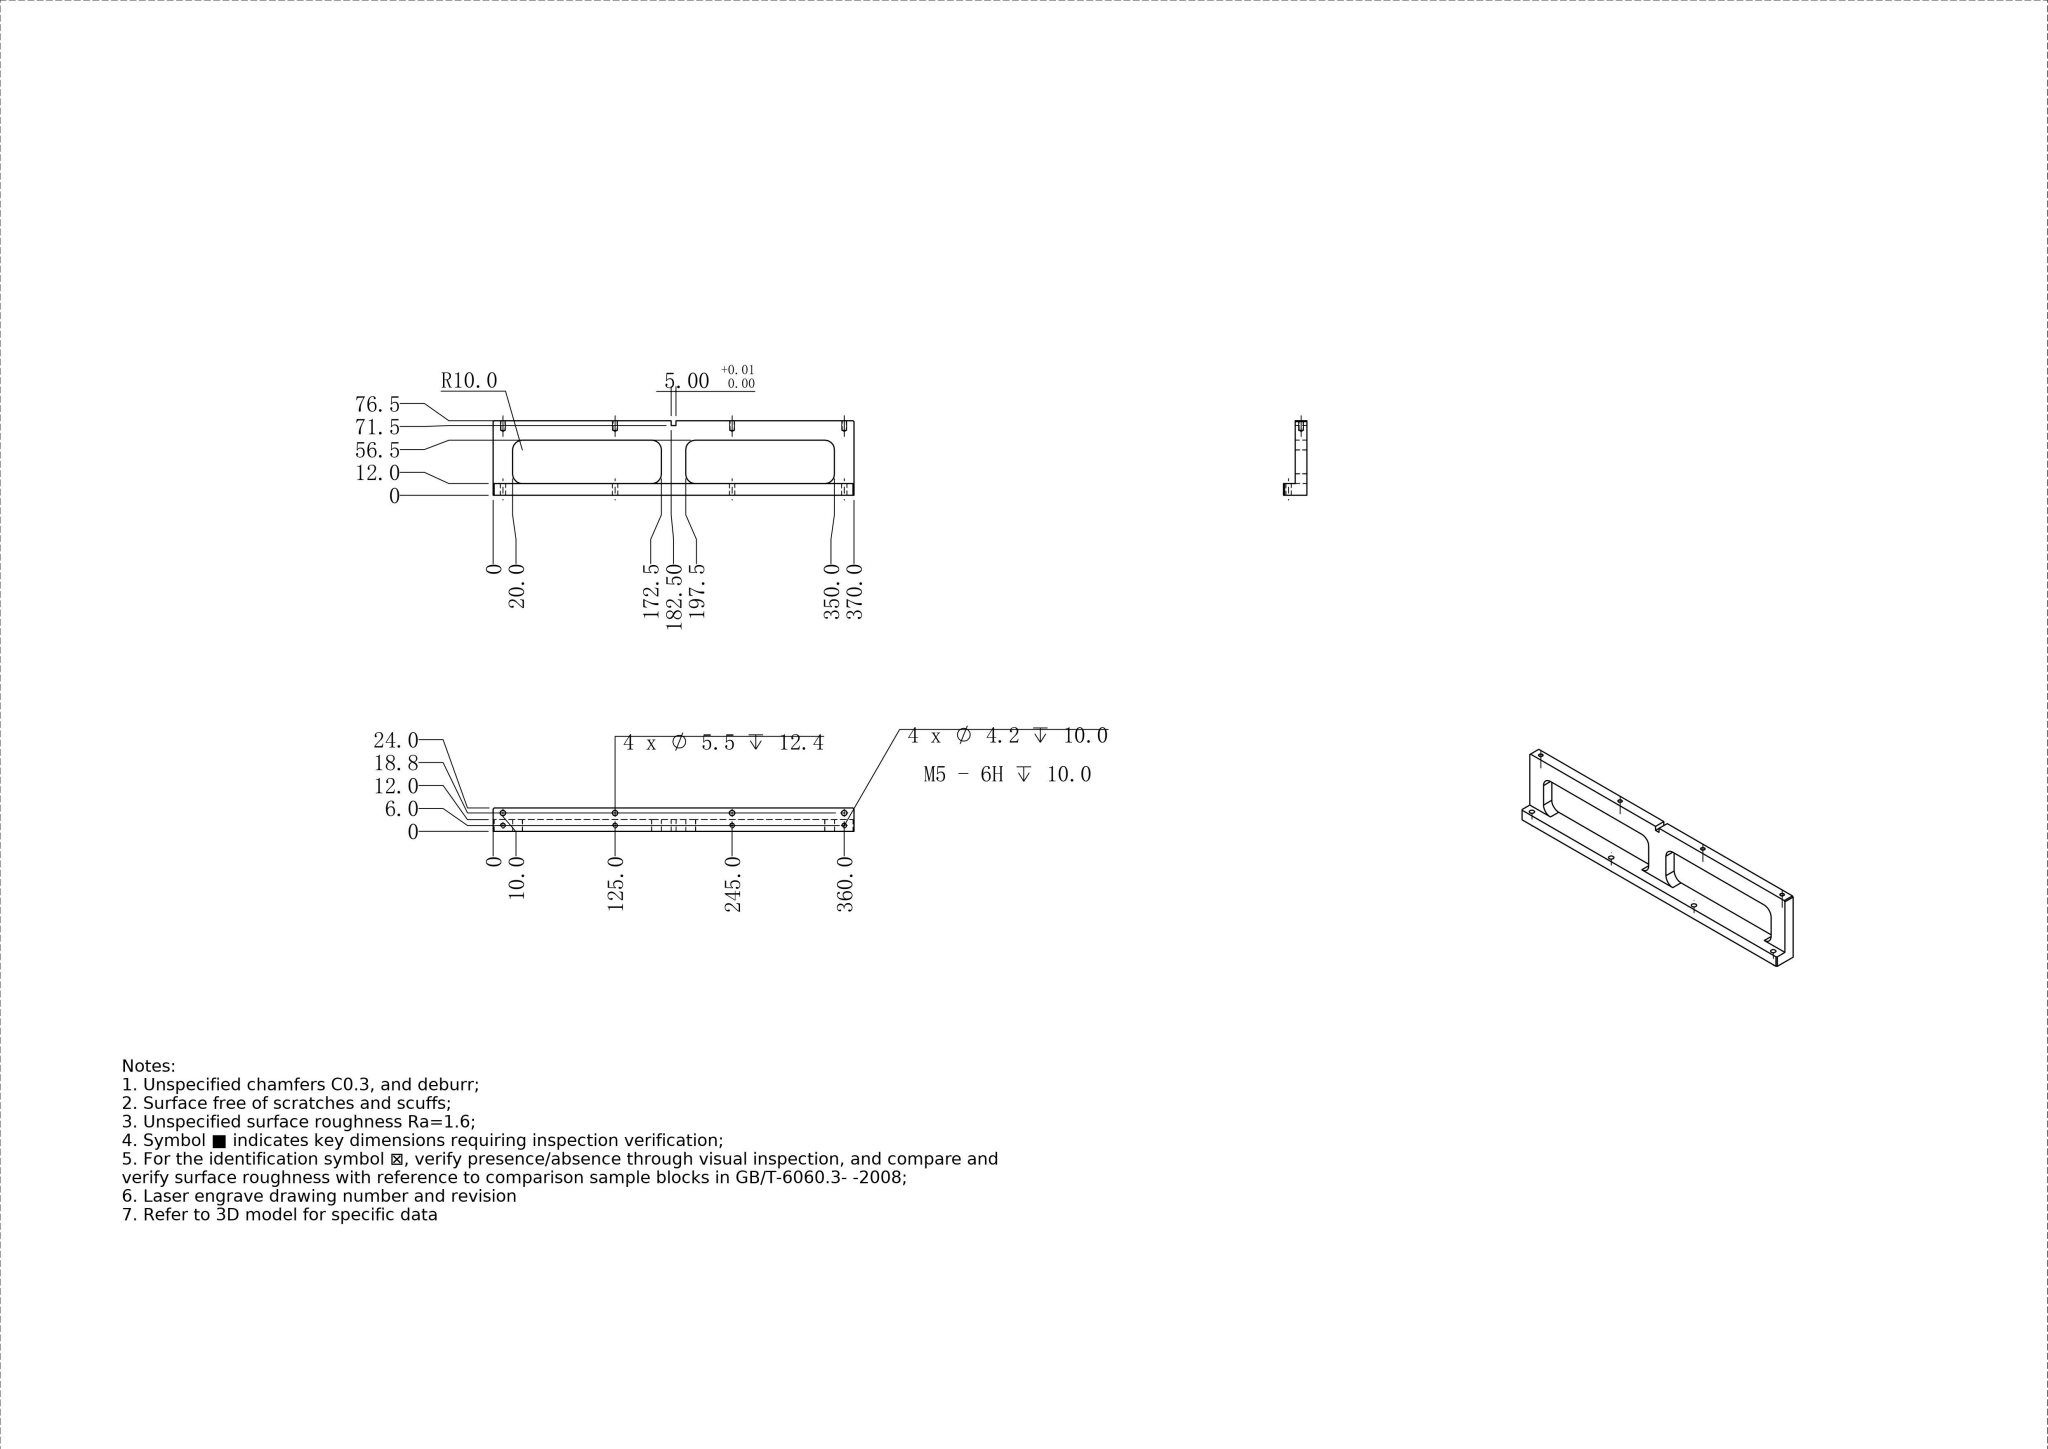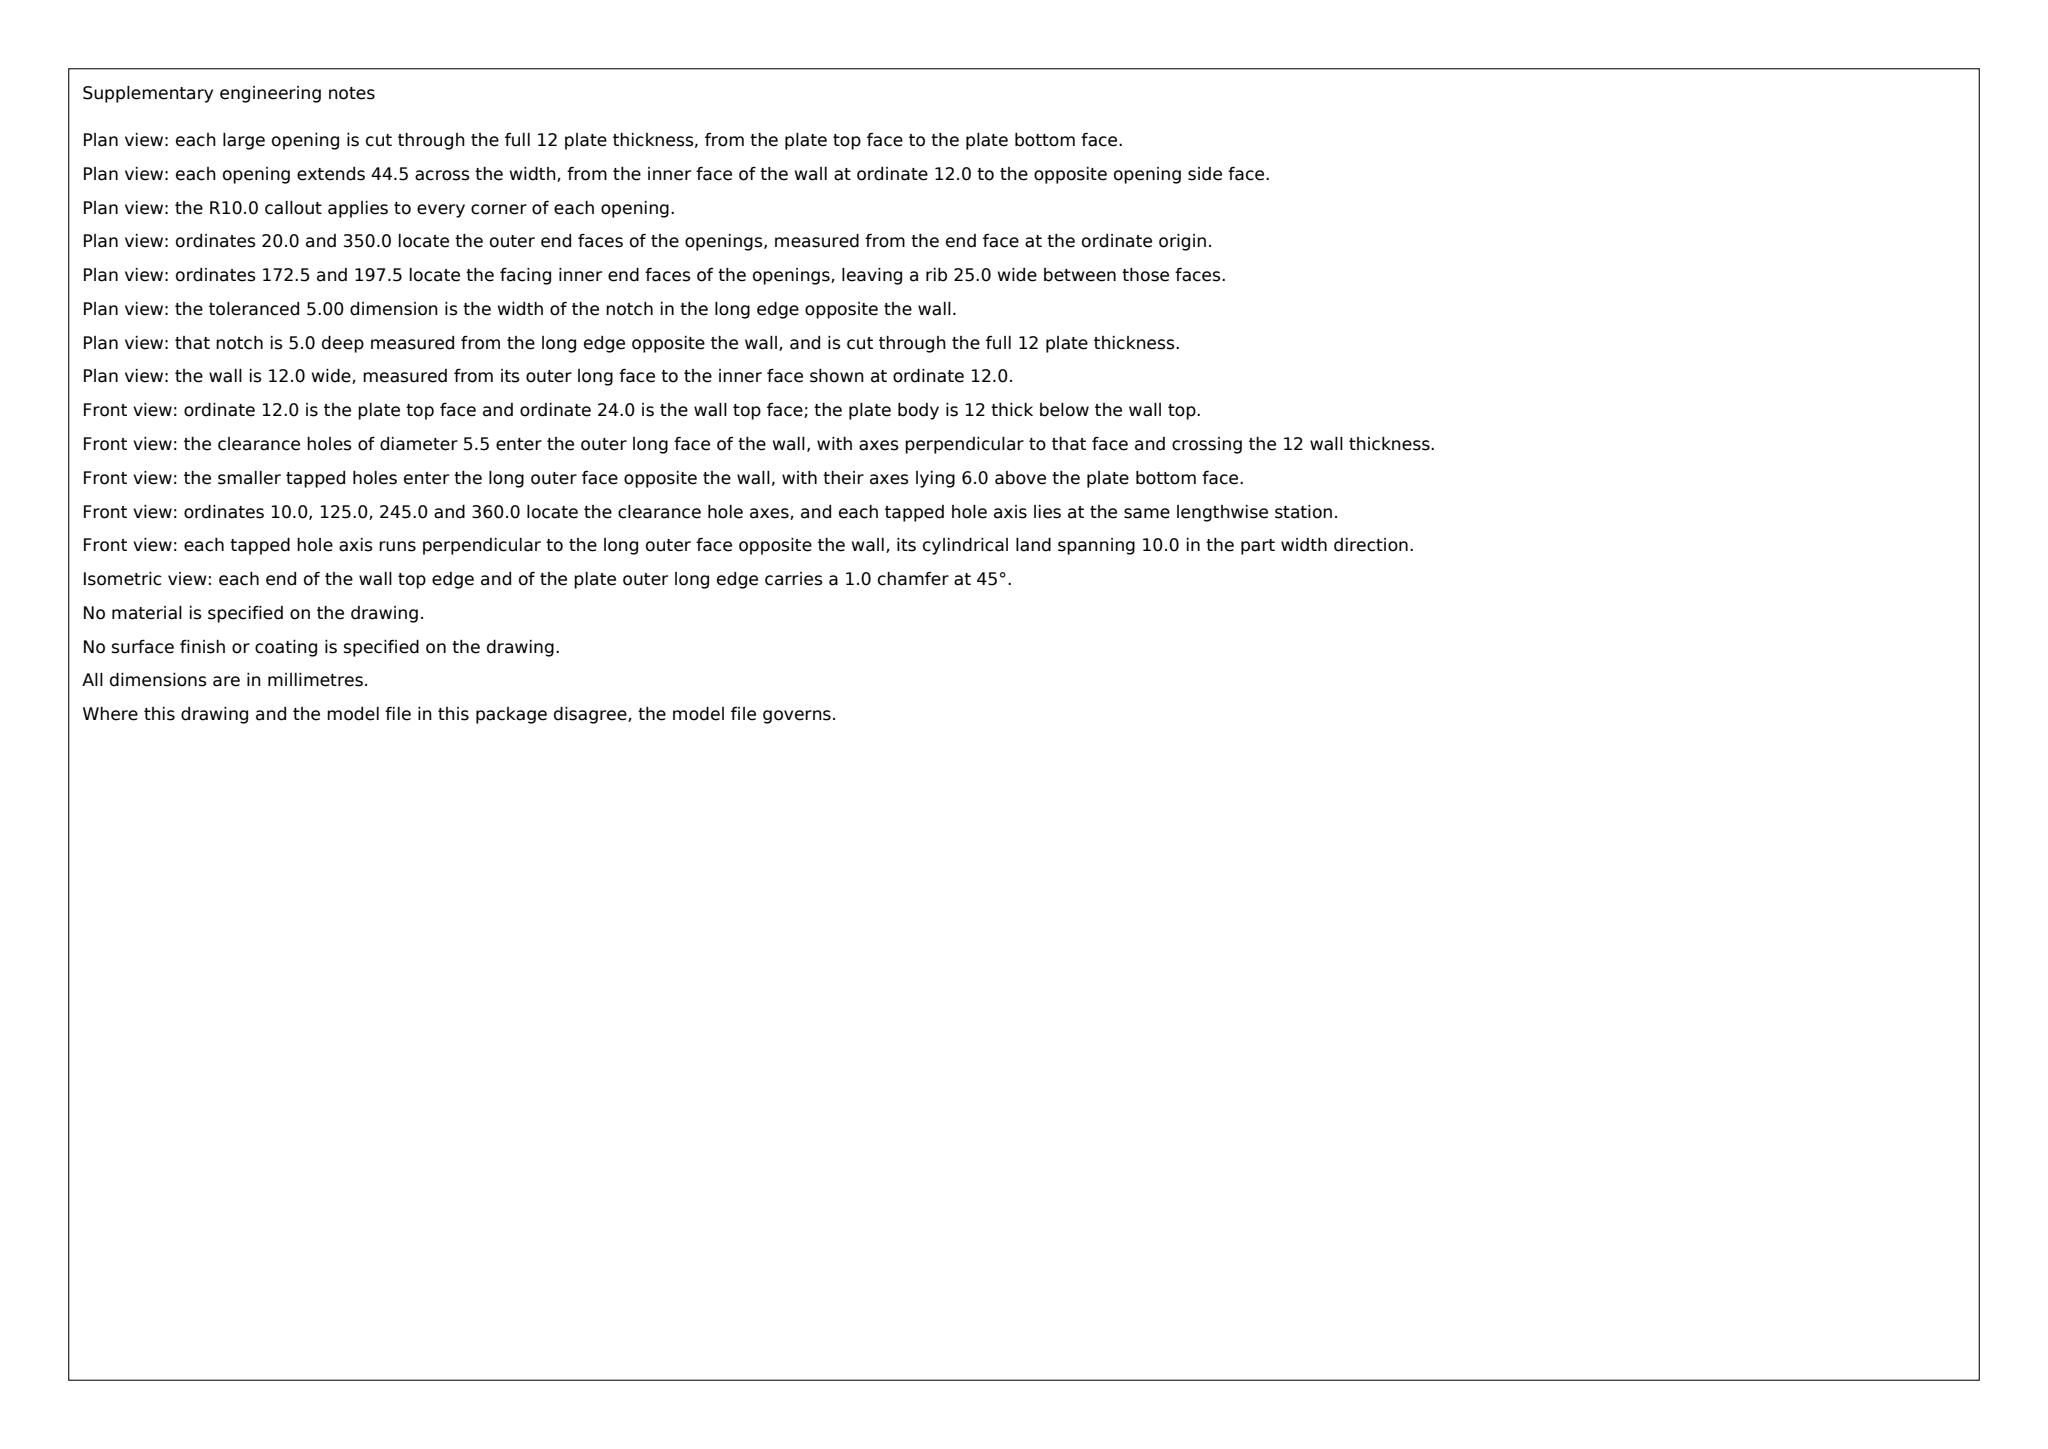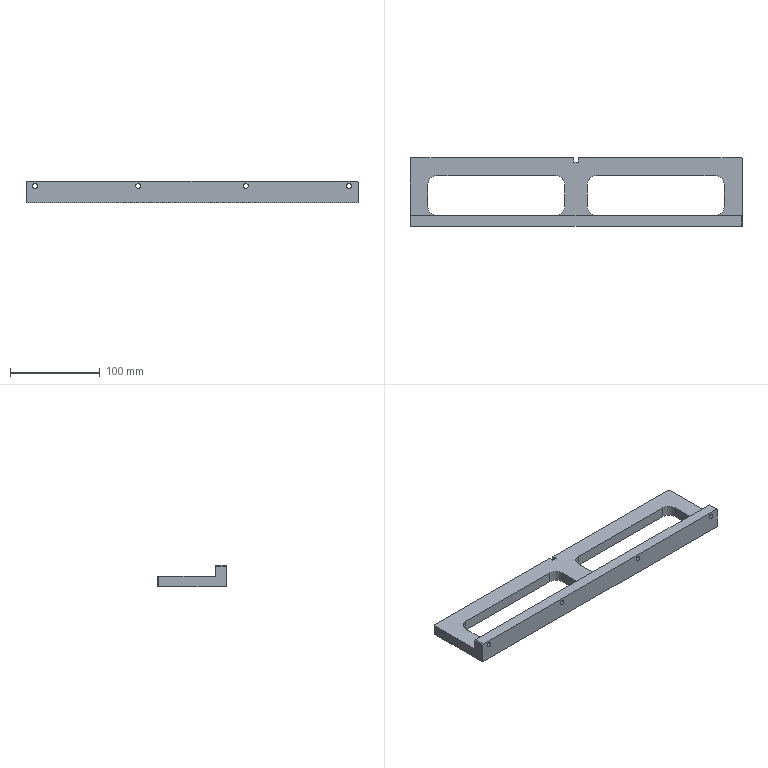Part | SolidWorks | mm | 1 solid | 54 faces | box 370 x 76.5 x 24 mm | volume 230088 mm3 | cylinder 24 | plane 22 | cone 8 | commonest cylinder face diameters 5.5 x8 4.2 x8 20 x8
build123d program:
from build123d import *

# Parameters (mm, degrees)
SKETCH1_W                = 370
SKETCH1_H                = 76.5
BOSS_EXTRUDE1_DEPTH      = 12
SKETCH2_W                = 370
SKETCH2_H                = 12
BOSS_EXTRUDE2_DEPTH      = 12
CHAMFER1_SIZE            = 1
SKETCH3_W                = 152.5
SKETCH3_H                = 44.5
CUT_EXTRUDE1_DEPTH       = 12
FILLET1_R                = 10
M5_TAPPED_HOLE4_D        = 4.2
M5_TAPPED_HOLE4_DEPTH    = 10
M5_TAPPED_HOLE4_TIP      = 1.262
SKETCH6_W                = 5
SKETCH6_H                = 10
CUT_EXTRUDE2_DEPTH       = 190.294
M5_CLEARANCE_HOLE1_D     = 5.5
M5_CLEARANCE_HOLE1_DEPTH = 12.4
M5_CLEARANCE_HOLE1_TIP   = 1.652


with BuildPart() as part:
    # Sketch1 → Boss-Extrude1 (new body)
    with BuildSketch(Plane.XY):
        Rectangle(SKETCH1_W, SKETCH1_H)
    extrude(amount=BOSS_EXTRUDE1_DEPTH)

    # Sketch2 → Boss-Extrude2 (add)
    with BuildSketch(Plane.XY.offset(12)):
        with Locations((0, -32.25)):
            Rectangle(SKETCH2_W, SKETCH2_H)
    extrude(amount=BOSS_EXTRUDE2_DEPTH)

    # Chamfer1
    chamfer1_edges = [part.edges().sort_by_distance(p)[0] for p in [
        (-185, -32.25, 24),
        (185, -32.25, 24),
        (-185, 38.25, 6),
        (185, 38.25, 6),
    ]]
    chamfer(chamfer1_edges, length=CHAMFER1_SIZE)

    # Sketch3 → Cut-Extrude1 (cut)
    with BuildSketch(Plane.XY.offset(12)):
        with Locations((-88.75, -4)):
            Rectangle(SKETCH3_W, SKETCH3_H)
        with Locations((88.75, -4)):
            Rectangle(SKETCH3_W, SKETCH3_H)
    extrude(amount=-CUT_EXTRUDE1_DEPTH, mode=Mode.SUBTRACT)

    # Fillet1
    fillet1_edges = [part.edges().sort_by_distance(p)[0] for p in [
        (-165, -26.25, 6),
        (-165, 18.25, 6),
        (-12.5, 18.25, 6),
        (-12.5, -26.25, 6),
        (12.5, -26.25, 6),
        (12.5, 18.25, 6),
        (165, 18.25, 6),
        (165, -26.25, 6),
    ]]
    fillet(fillet1_edges, radius=FILLET1_R)

    # M5 Tapped Hole4
    with Locations(Plane(origin=(0, 38.25, 0), x_dir=(1, 0, 0), z_dir=(0, 1, 0))):
        with Locations((-175, -6), (-60, -6), (60, -6), (175, -6)):
            Hole(M5_TAPPED_HOLE4_D / 2, depth=M5_TAPPED_HOLE4_DEPTH)
            with Locations((0, 0, -(M5_TAPPED_HOLE4_DEPTH + M5_TAPPED_HOLE4_TIP / 2))):  # 118° drill point
                Cone(0, M5_TAPPED_HOLE4_D / 2, M5_TAPPED_HOLE4_TIP, mode=Mode.SUBTRACT)

    # Sketch6 → Cut-Extrude2 (cut, through all)
    with BuildSketch(Plane.XY.offset(12)):
        with Locations((0, 38.25)):
            Rectangle(SKETCH6_W, SKETCH6_H)
    extrude(amount=-CUT_EXTRUDE2_DEPTH, mode=Mode.SUBTRACT)

    # M5 Clearance Hole1
    with Locations(Plane(origin=(0, -26.25, 0), x_dir=(1, 0, 0), z_dir=(0, 1, 0))):
        with Locations((-175, -18.837), (-60, -18.837), (60, -18.837), (175, -18.837)):
            Hole(M5_CLEARANCE_HOLE1_D / 2, depth=M5_CLEARANCE_HOLE1_DEPTH)
            with Locations((0, 0, -(M5_CLEARANCE_HOLE1_DEPTH + M5_CLEARANCE_HOLE1_TIP / 2))):  # 118° drill point
                Cone(0, M5_CLEARANCE_HOLE1_D / 2, M5_CLEARANCE_HOLE1_TIP, mode=Mode.SUBTRACT)


solid = part.part